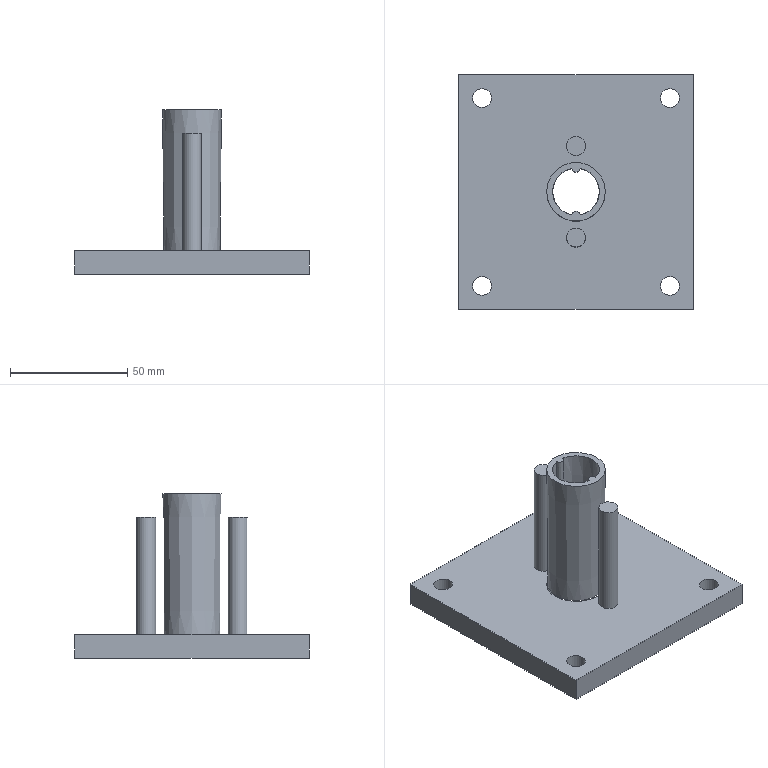Component | NX | DIE1 | 2 solids | 22 faces | volume 106968 mm3 | plane 10 | cylinder 7 | cone 5 | commonest cylinder face diameters 8 x6 25 x1